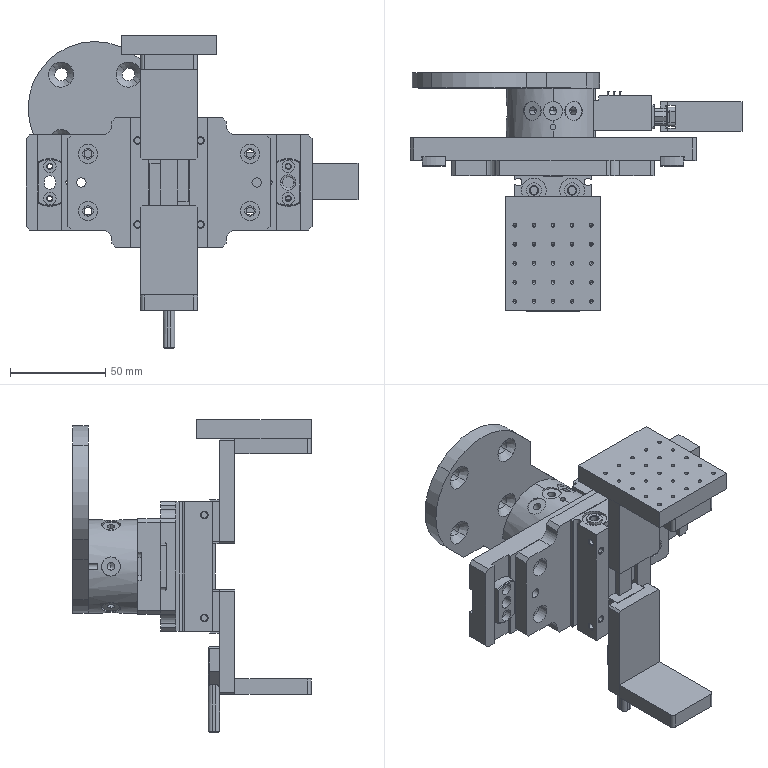Assembly | SolidWorks | mm | 15 component files | 17 solids | 1284 faces | box 174.1 x 125 x 164 mm | volume 368632 mm3 | cylinder 576 | plane 512 | cone 192 | spline 4 | commonest cylinder face diameters 1 x90 2 x84 10 x42 1.06 x38 2.459 x28 4.134 x26 3 x24 6 x24
Bill of materials:
F-JBEH10-P7-W6-L8 | 1 |  | Thick plate with two straight sides and two convex arc ends, and a stepped cylindrical boss on one face. The plate has two small round through-holes and an elongated (obround) central through-opening.
F-JBNF10-P6-L8 | 1 |  | Thick plate with two straight sides and two convex arc ends, and a stepped cylindrical boss on one face. The plate has two small round through-holes and a round central hole with a chamfered or counterbored ring around it.
F-SCHUNK-0301265 KAS-A15-A | 1 |  | Long rectangular block body with a thin plate flange across it near one end. The flange sticks out past the body and has a round hole in each extended tab. A shorter rectangular section with rounded edges extends beyond the flange.
F-_SCHUNK-SWA 005-000-000-parts, 01 | 1 |  | Short cylindrical housing with a large central through-bore and a thin rod running across the bore. A flat rectangular pad is raised on one side. The part has several holes: four through-holes in the end face, counterbored or spot-faced holes on the curved surface, small conical-bottom holes on the side pad, and two dome-ended studs that protrude.
F-SCHUNK-9937327 SWO-B15-A | 1 |  | Rectangular box body. One face has a trapezoidal (D-shaped) raised shroud containing a grid of small holes, with a hex standoff carrying a hole on each side of it. Two cylindrical pins project from the opposite end. Rows of thin pins stick out from one side face, and the large face has two shallow conical recesses.
F-SZP17248-10-03 | 1 |  | Long rectangular plate with chamfered corners and a symmetric pattern of round through-holes of several sizes. A raised step or boss runs along one face, and there are shallow notches or recesses on the opposite face near the ends.
F-SZP17248-10-04 | 1 |  | Flat plate of uniform thickness. Its outline is a rectangle with chamfered corners, and a wider central section with concave rounded notches where it steps down to narrower end tabs. Each end tab has three round through-holes in a vertical line: two larger holes and one smaller middle hole.
F-SZP17248-10-11 | 1 |  | Flat plate of uniform thickness with a dog-bone-like outline: a large rounded lobe joined at an angle to an elongated arm with a rounded end. The lobe has four countersunk through-holes in a square pattern. The arm has two medium holes and several small holes.
GripperJaw1 | 2 | 1060 Alloy | Plain rectangular block or thick plate with small chamfers on the corners. No holes or other features are visible.
GripperJaw2 | 2 | 1060 Alloy | Rectangular plate or slab with rounded vertical corners, at least on two adjacent corners. No holes or other features are visible.
GripperJaw3 | 1 |  | Flat plate head shaped like a pentagon or shield, with chamfered top corners, two round through-holes, and a tapered lower edge. A straight shaft with a rounded or chamfered end extends from the point of the taper.
LabelSuctionPlate | 1 |  | Rectangular block or thick plate with a regular 5 by 5 grid of 25 small holes on one face.
MHF2-12D1_24_0 | 1 |  | Elongated, roughly rectangular prismatic block with a stepped, T-like cross-section. One long face has two raised pads, one at each end, with a recessed channel between them. The block is drilled with several counterbored and plain holes. There is a semicircular lengthwise groove along each side edge, and a narrow longitudinal groove runs along one side face.
Mates:
1. concentric | F-SWS-005-000-000-1/F-SCHUNK-0302308 SWA-005-000-000, 00-1/F-_SCHUNK-SWA 005-000-000-parts, 01-1 face at (-45.188, -18.343, 123.72) dir (0, 1, 0) r 12.5 | F-SZP17248-10-03-1 face at (-45.188, -15.343, 123.72) dir (0, -1, 0) r 12.5
2. concentric | F-SWS-005-000-000-1/F-SCHUNK-0302308 SWA-005-000-000, 00-1/F-_SCHUNK-SWA 005-000-000-parts, 01-1 face at (-25.188, -18.343, 123.72) dir (0, 1, 0) r 1.5 | F-SZP17248-10-03-1 face at (-25.188, -15.343, 123.72) dir (0, -1, 0) r 1.5
3. coincident | F-SWS-005-000-000-1/F-SCHUNK-0302308 SWA-005-000-000, 00-1/F-_SCHUNK-SWA 005-000-000-parts, 01-1 face at (-32.688, -18.343, 123.72) dir (0, -1, 0) | F-SZP17248-10-03-1 face at (-45.188, -18.343, 123.72) dir (0, 1, 0)
4. concentric | F-SZP17248-10-03-1 face at (-107.688, -30.343, 123.72) dir (0, 1, 0) r 5 | F-JBEH10-P7-W6-L8-1 face at (-107.688, -20.343, 123.72) dir (0, -1, 0) r 5
5. concentric | F-SZP17248-10-03-1 face at (17.312, -30.343, 123.72) dir (0, 1, 0) r 5 | F-JBNF10-P6-L8-1 face at (17.312, -20.343, 123.72) dir (0, -1, 0) r 5
6. coincident | F-SZP17248-10-03-1 face at (-45.188, -30.343, 123.72) dir (0, -1, 0) | F-SZP17248-10-04-1 face at (-45.188, -30.343, 123.72) dir (0, 1, 0)
7. width | F-SZP17248-10-04-1 face at (7.812, -30.343, 148.72) dir (1, 0, 0) | F-SZP17248-10-04-1 face at (-98.188, -30.343, 148.72) dir (-1, 0, 0) | F-SZP17248-10-03-1 face at (29.812, -18.343, 148.72) dir (1, 0, 0) | F-SZP17248-10-03-1 face at (-120.188, -18.343, 148.72) dir (-1, 0, 0)
8. width | F-SZP17248-10-04-1 face at (7.812, -30.343, 98.72) dir (0, 0, -1) | F-SZP17248-10-04-1 face at (7.812, -30.343, 148.72) dir (0, 0, 1) | F-SZP17248-10-03-1 face at (-120.188, -18.343, 98.72) dir (0, 0, -1) | F-SZP17248-10-03-1 face at (-120.188, -18.343, 148.72) dir (0, 0, 1)
9. coincident | F-SZP17248-10-03-1 face at (-45.188, -28.343, 123.72) dir (0, -1, 0) | F-JBNF10-P6-L8-1 face at (17.312, -28.343, 119.22) dir (0, 1, 0)
10. parallel | F-SZP17248-10-03-1 face at (23.562, -28.343, 123.72) dir (-1, 0, 0) | F-JBNF10-P6-L8-1 face at (23.312, -28.343, 136.22) dir (1, 0, 0)
11. coincident | F-SZP17248-10-03-1 face at (-45.188, -28.343, 123.72) dir (0, -1, 0) | F-JBEH10-P7-W6-L8-1 face at (-107.688, -28.343, 136.22) dir (0, 1, 0)
12. parallel | F-SZP17248-10-03-1 face at (-113.938, -28.343, 123.72) dir (1, 0, 0) | F-JBEH10-P7-W6-L8-1 face at (-113.688, -28.343, 136.22) dir (-1, 0, 0)
13. concentric | assembly face at (-45.188, 25.157, 123.72) dir (0, 1, 0) r 24.5 | F-SZP17248-10-11-1 face at (-45.188, 7.657, 123.72) dir (0, 1, 0) r 24.5
14. coincident | assembly face at (-45.188, 33.157, 123.72) dir (0, 1, 0) | F-SZP17248-10-11-1 face at (-45.188, 7.657, 123.72) dir (0, -1, 0)
15. coincident | F-SZP17248-10-04-1 face at (-45.188, -38.343, 123.72) dir (0, -1, 0) | MHF2-12D1_24_0-1 face at (-50.488, -38.343, 157.72) dir (0, 1, 0)
16. coincident | F-SZP17248-10-04-1 face at (-45.188, -34.343, 89.72) dir (0, 0, -1) | MHF2-12D1_24_0-1 face at (-45.188, -38.343, 89.72) dir (0, 0, -1)
17. width | MHF2-12D1_24_0-1 face at (-25.188, -57.343, 157.72) dir (1, 0, 0) | MHF2-12D1_24_0-1 face at (-65.188, -43.143, 157.72) dir (-1, 0, 0) | F-SZP17248-10-04-1 face at (-98.188, -30.343, 148.72) dir (-1, 0, 0) | F-SZP17248-10-04-1 face at (7.812, -30.343, 148.72) dir (1, 0, 0)
18. coincident | MHF2-12D1_24_0-1 face at (-49.188, -63.343, 135.72) dir (0, -1, 0) | GripperJaw1-1 face at (-45.188, -63.343, 163.22) dir (0, 1, 0)
19. coincident | MHF2-12D1_24_0-1 face at (-45.188, -63.343, 135.72) dir (0, 0, -1) | GripperJaw1-1 face at (-60.188, -61.343, 135.72) dir (0, 0, -1)
20. width | GripperJaw1-1 face at (-30.188, -61.343, 135.72) dir (1, 0, 0) | GripperJaw1-1 face at (-60.188, -61.343, 135.72) dir (-1, 0, 0) | MHF2-12D1_24_0-1 face at (-55.188, -63.343, 135.72) dir (-1, 0, 0) | MHF2-12D1_24_0-1 face at (-35.188, -53.543, 135.72) dir (1, 0, 0)
21. coincident | MHF2-12D1_24_0-1 face at (-41.188, -63.343, 111.72) dir (0, -1, 0) | GripperJaw1-2 face at (-45.188, -63.343, 84.22) dir (0, 1, 0)
22. coincident | MHF2-12D1_24_0-1 face at (-45.188, -63.343, 111.72) dir (0, 0, 1) | GripperJaw1-2 face at (-30.188, -61.343, 111.72) dir (0, 0, 1)
23. width | GripperJaw1-2 face at (-60.188, -61.343, 111.72) dir (-1, 0, 0) | GripperJaw1-2 face at (-30.188, -61.343, 111.72) dir (1, 0, 0) | MHF2-12D1_24_0-1 face at (-35.188, -63.343, 111.72) dir (1, 0, 0) | MHF2-12D1_24_0-1 face at (-55.188, -53.543, 111.72) dir (-1, 0, 0)
24. coincident | GripperJaw1-1 face at (-45.188, -69.343, 163.22) dir (0, -1, 0) | GripperJaw2-1 face at (-60.188, -69.343, 190.72) dir (0, 1, 0)
25. coincident | GripperJaw1-1 face at (-60.188, -61.343, 190.72) dir (0, 0, 1) | GripperJaw2-1 face at (-45.188, -89.343, 190.72) dir (0, 0, 1)
26. coincident | GripperJaw1-1 face at (-60.188, -61.343, 135.72) dir (-1, 0, 0) | GripperJaw2-1 face at (-60.188, -69.343, 190.72) dir (-1, 0, 0)
27. coincident | GripperJaw1-2 face at (-45.188, -69.343, 84.22) dir (0, -1, 0) | GripperJaw2-2 face at (-60.188, -69.343, 64.72) dir (0, 1, 0)
28. coincident | GripperJaw1-2 face at (-60.188, -61.343, 111.72) dir (-1, 0, 0) | GripperJaw2-2 face at (-60.188, -69.343, 64.72) dir (-1, 0, 0)
29. coincident | GripperJaw1-2 face at (-30.188, -61.343, 56.72) dir (0, 0, -1) | GripperJaw2-2 face at (-45.188, -89.343, 56.72) dir (0, 0, -1)
30. coincident | GripperJaw1-2 face at (-45.188, -61.343, 84.22) dir (0, 1, 0) | GripperJaw3-1 face at (-45.188, -61.343, 59.22) dir (0, -1, 0)
31. width | GripperJaw3-1 face at (-35.188, -55.343, 81.72) dir (1, 0, 0) | GripperJaw3-1 face at (-55.188, -55.343, 81.72) dir (-1, 0, 0) | GripperJaw1-2 face at (-60.188, -61.343, 111.72) dir (-1, 0, 0) | GripperJaw1-2 face at (-30.188, -61.343, 111.72) dir (1, 0, 0)
32. distance | GripperJaw3-1 face at (-55.188, -55.343, 81.72) dir (0, 0, 1) | GripperJaw1-2 face at (-30.188, -61.343, 56.72) dir (0, 0, -1)
33. coincident | GripperJaw2-1 face at (-45.188, -89.343, 190.72) dir (0, 0, 1) | LabelSuctionPlate-1 face at (-45.188, -79.343, 190.72) dir (0, 0, -1)
34. coincident | GripperJaw2-1 face at (-60.188, -109.343, 190.72) dir (0, -1, 0) | LabelSuctionPlate-1 face at (-70.188, -109.343, 200.72) dir (0, -1, 0)
35. width | LabelSuctionPlate-1 face at (-70.188, -49.343, 200.72) dir (-1, 0, 0) | LabelSuctionPlate-1 face at (-20.188, -49.343, 200.72) dir (1, 0, 0) | GripperJaw2-1 face at (-30.188, -69.343, 190.72) dir (1, 0, 0) | GripperJaw2-1 face at (-60.188, -69.343, 190.72) dir (-1, 0, 0)
36. coincident | F-SWS-005-000-000-1/F-SCHUNK-0302308 SWA-005-000-000, 00-1/F-_SCHUNK-SWA 005-000-000-parts, 01-1 face at (-20.688, 7.657, 123.72) dir (0, 1, 0) | F-SZP17248-10-11-1 face at (-45.188, 7.657, 123.72) dir (0, -1, 0)
37. concentric | F-SCHUNK-0302308 SWA-005-000-000, 00-1/F-_SCHUNK-SWA 005-000-000-parts, 01-1 face at (21, -11, -10) dir (-1, 0, 0) r 1.23 | F-SCHUNK-9937327 SWO-B15-A-1 face at (21.001, -11, -10) dir (-1, 0, 0) r 1.5
38. concentric | F-SCHUNK-0302308 SWA-005-000-000, 00-1/F-_SCHUNK-SWA 005-000-000-parts, 01-1 face at (21, -11, 10) dir (-1, 0, 0) r 1.23 | F-SCHUNK-9937327 SWO-B15-A-1 face at (21.001, -11, 10) dir (-1, 0, 0) r 1.5
39. coincident | F-SCHUNK-0302308 SWA-005-000-000, 00-1/F-_SCHUNK-SWA 005-000-000-parts, 01-1 face at (21, 0.009, 7) dir (1, 0, 0) | F-SCHUNK-9937327 SWO-B15-A-1 face at (21, -3.9, 7.5) dir (-1, 0, 0)
40. concentric | F-SCHUNK-9937327 SWO-B15-A-1 face at (59.4, -15, 12.5) dir (-1, 0, 0) r 1.23 | F-SCHUNK-0301265 KAS-A15-A-1 face at (58.9, -15, 12.5) dir (-1, 0, 0) r 1.6
41. parallel | F-SCHUNK-9937327 SWO-B15-A-1 face at (21, -22.2, -15.5) dir (0, -1, 0) | F-SCHUNK-0301265 KAS-A15-A-1 face at (99.1, -22.75, 0.5) dir (0, -1, 0)
42. coincident | F-SCHUNK-9937327 SWO-B15-A-1 face at (59.3, -22.2, -15.5) dir (1, 0, 0) | F-SCHUNK-0301265 KAS-A15-A-1 face at (59.3, -7.25, 0.5) dir (-1, 0, 0)